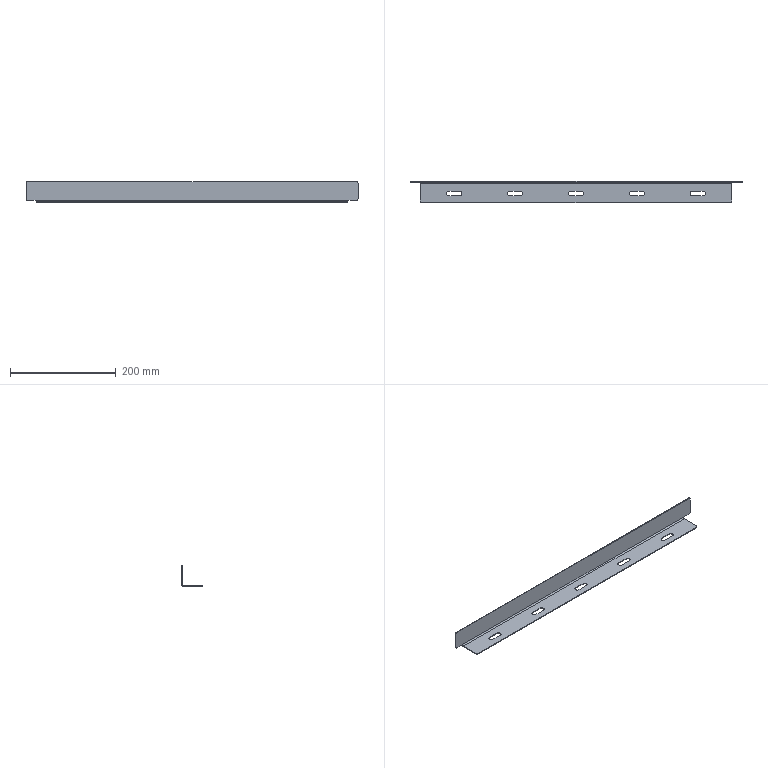Component | SolidWorks | FrameLongitudinalBeamOne01100-2 | 1 solid | 42 faces | volume 67860 mm3 | plane 24 | cylinder 18 | commonest cylinder face diameters 9 x10 6 x6 8 x1 5 x1